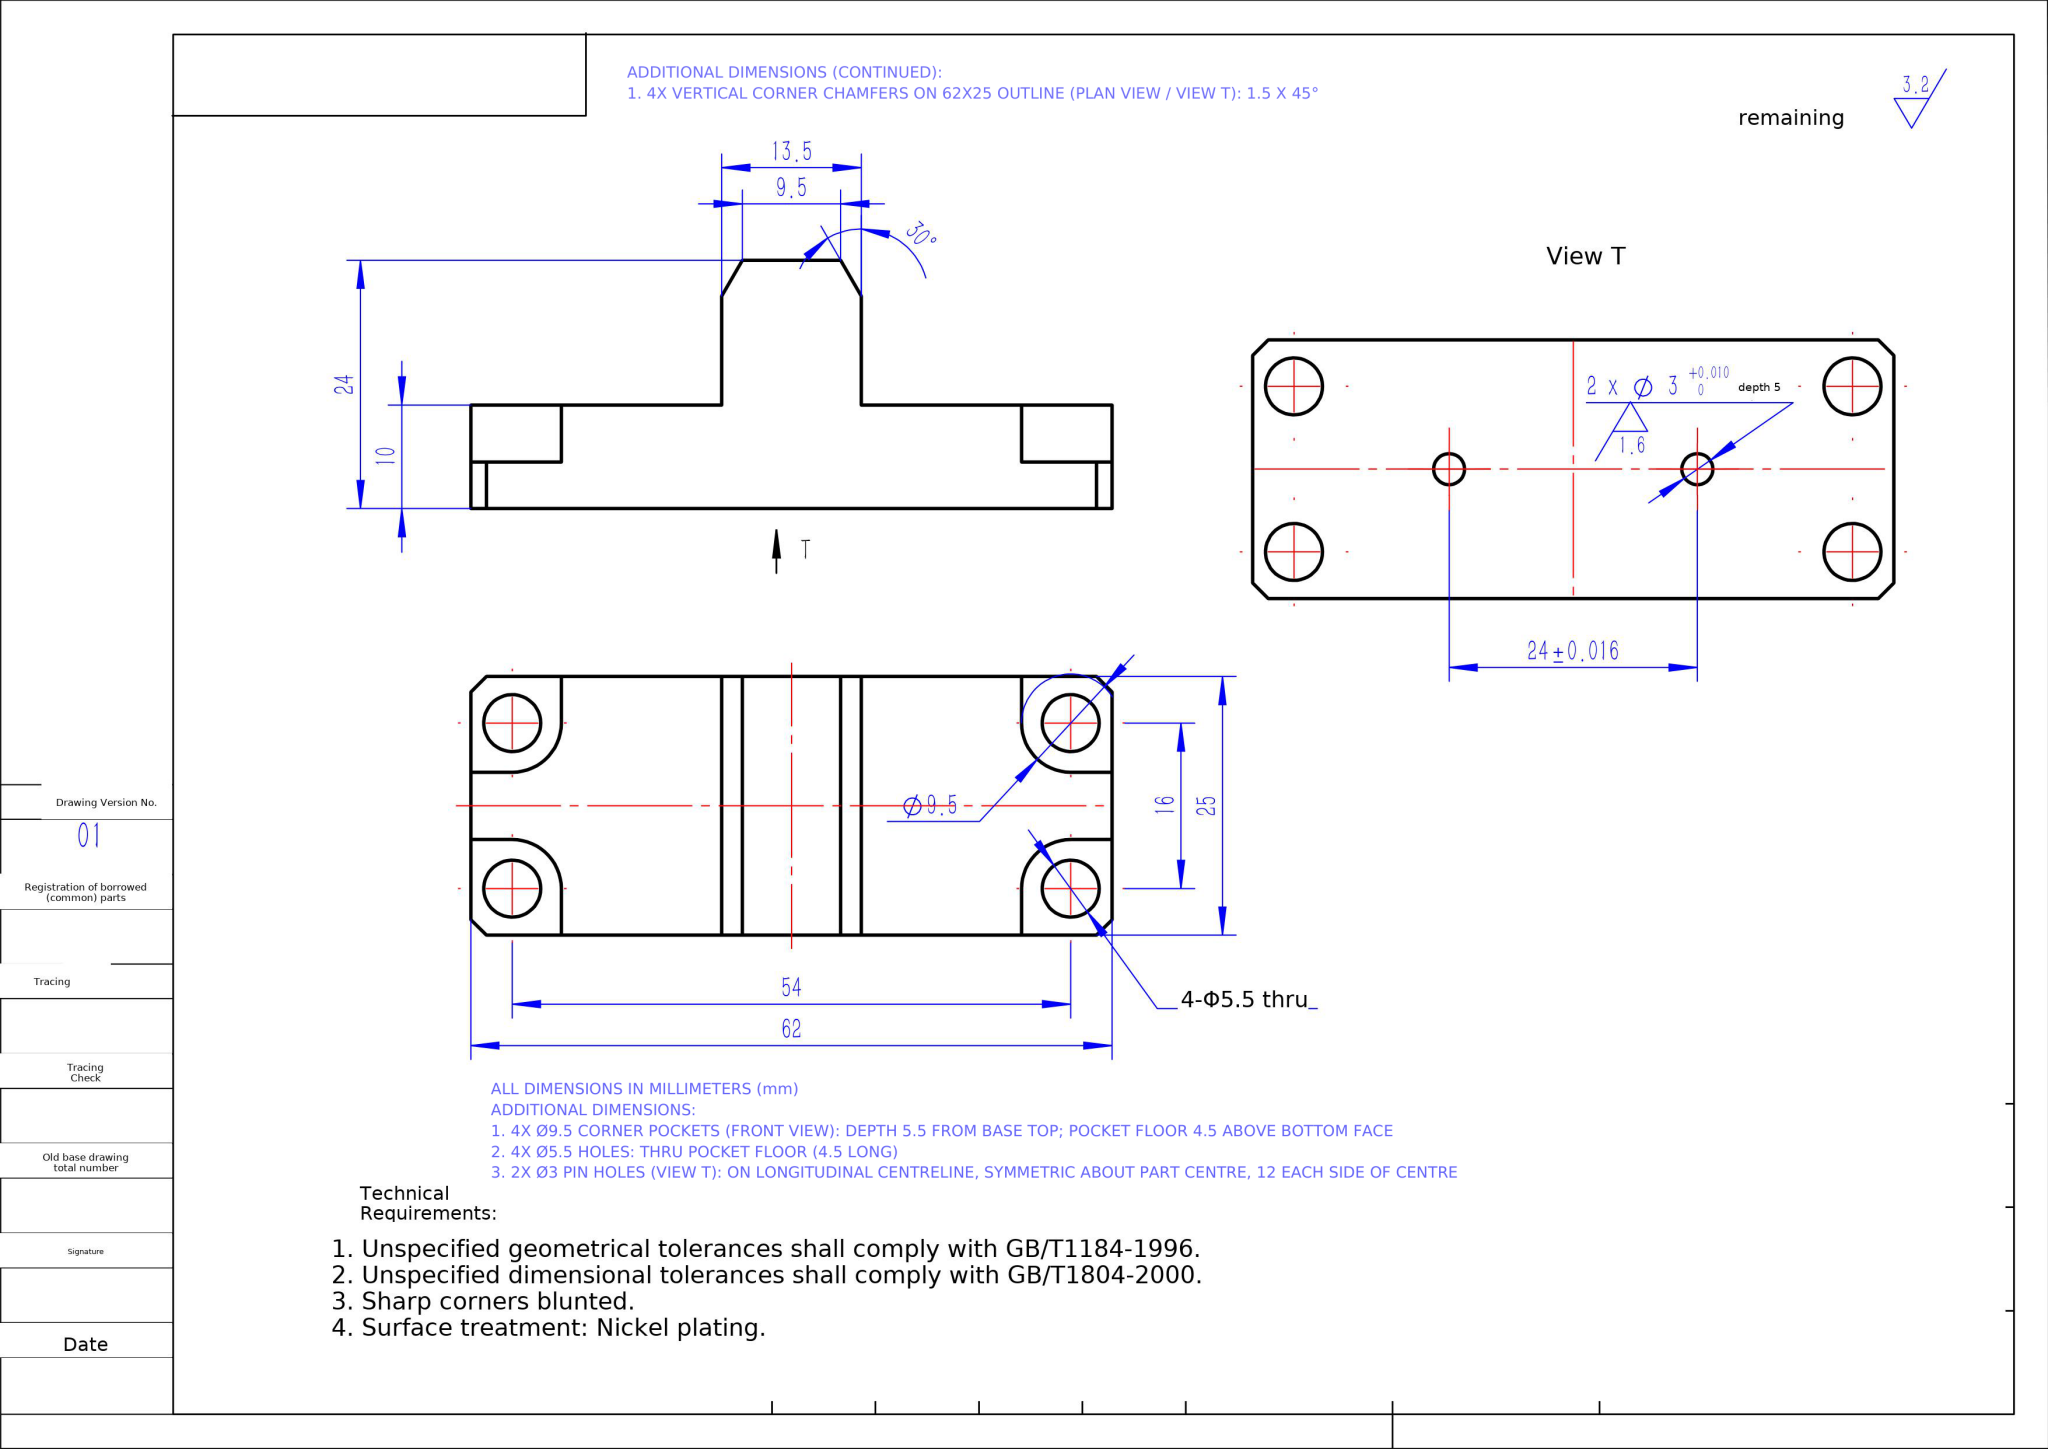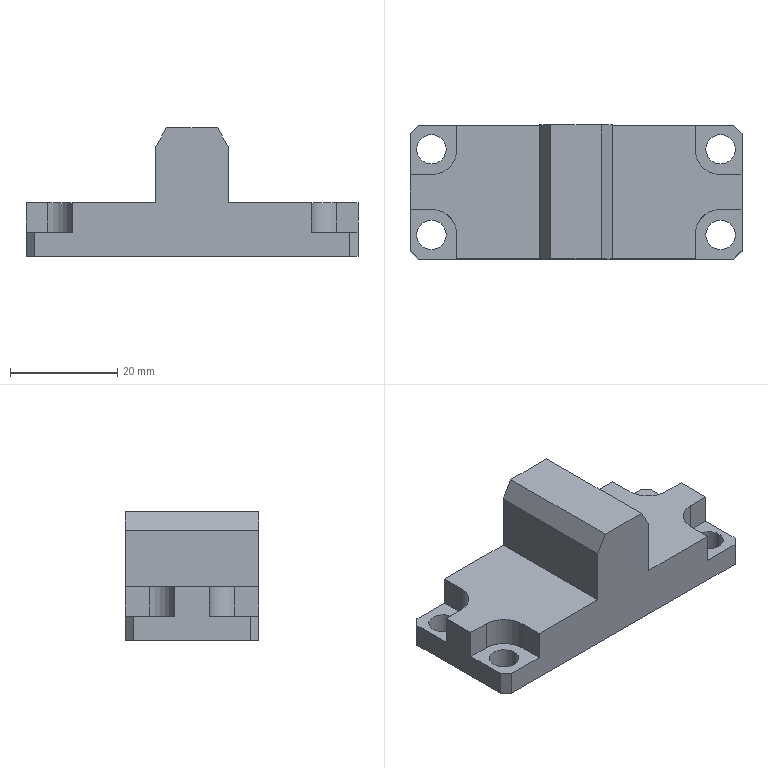Part | NX | mm | 1 solid | 48 faces | box 62 x 25 x 24 mm | volume 17855 mm3 | plane 28 | cylinder 16 | cone 4 | commonest cylinder face diameters 5.5 x8 3 x4 9.5 x4